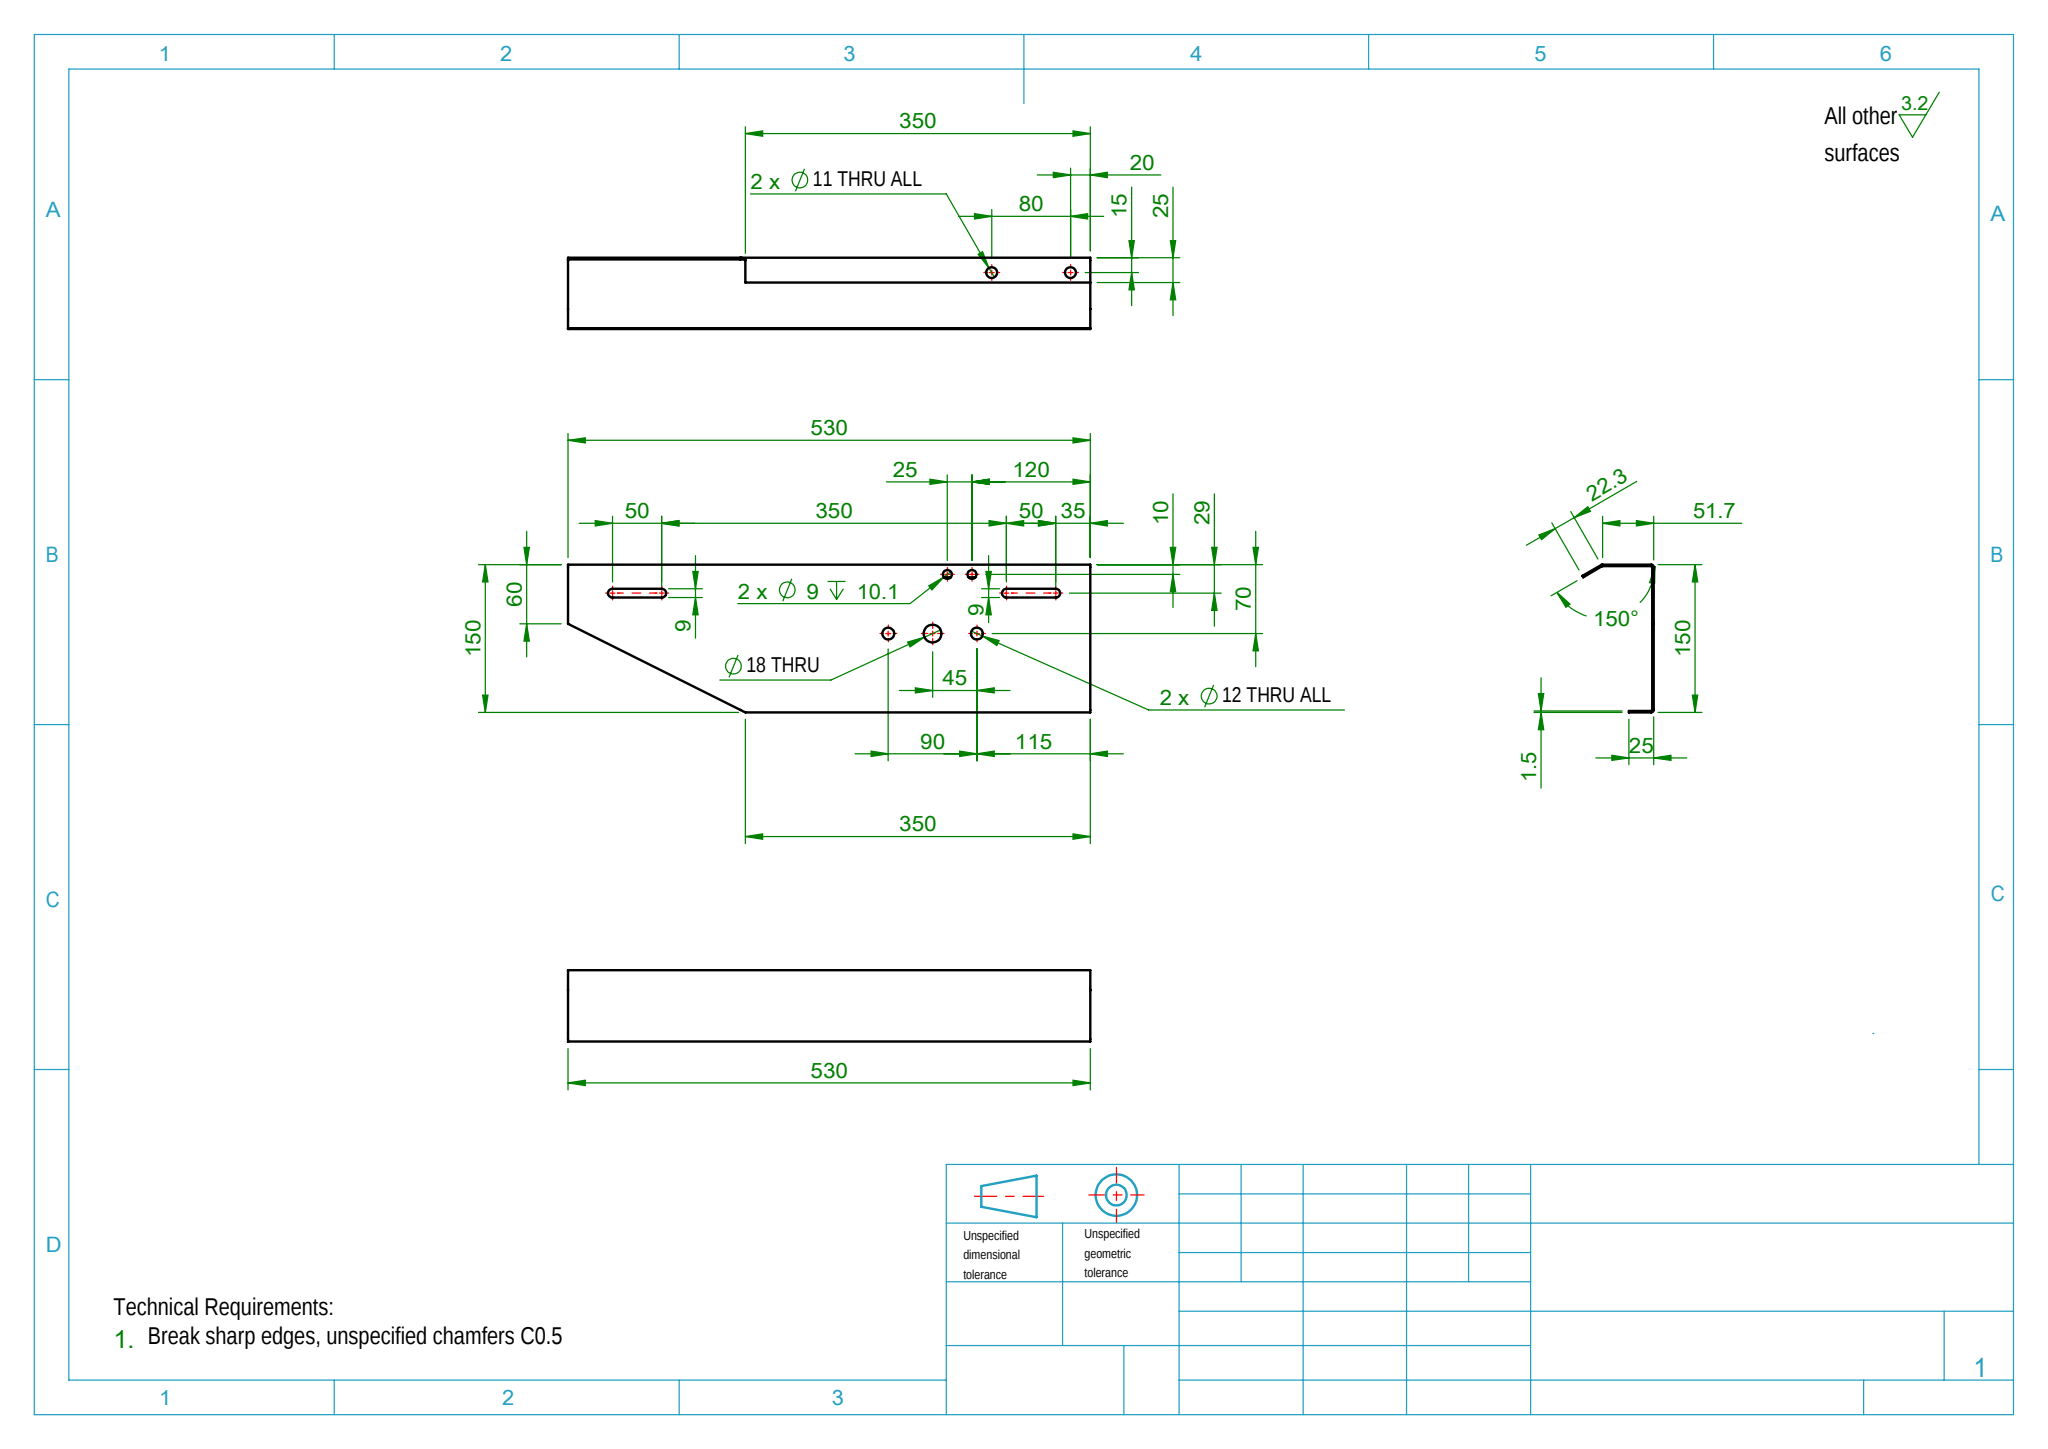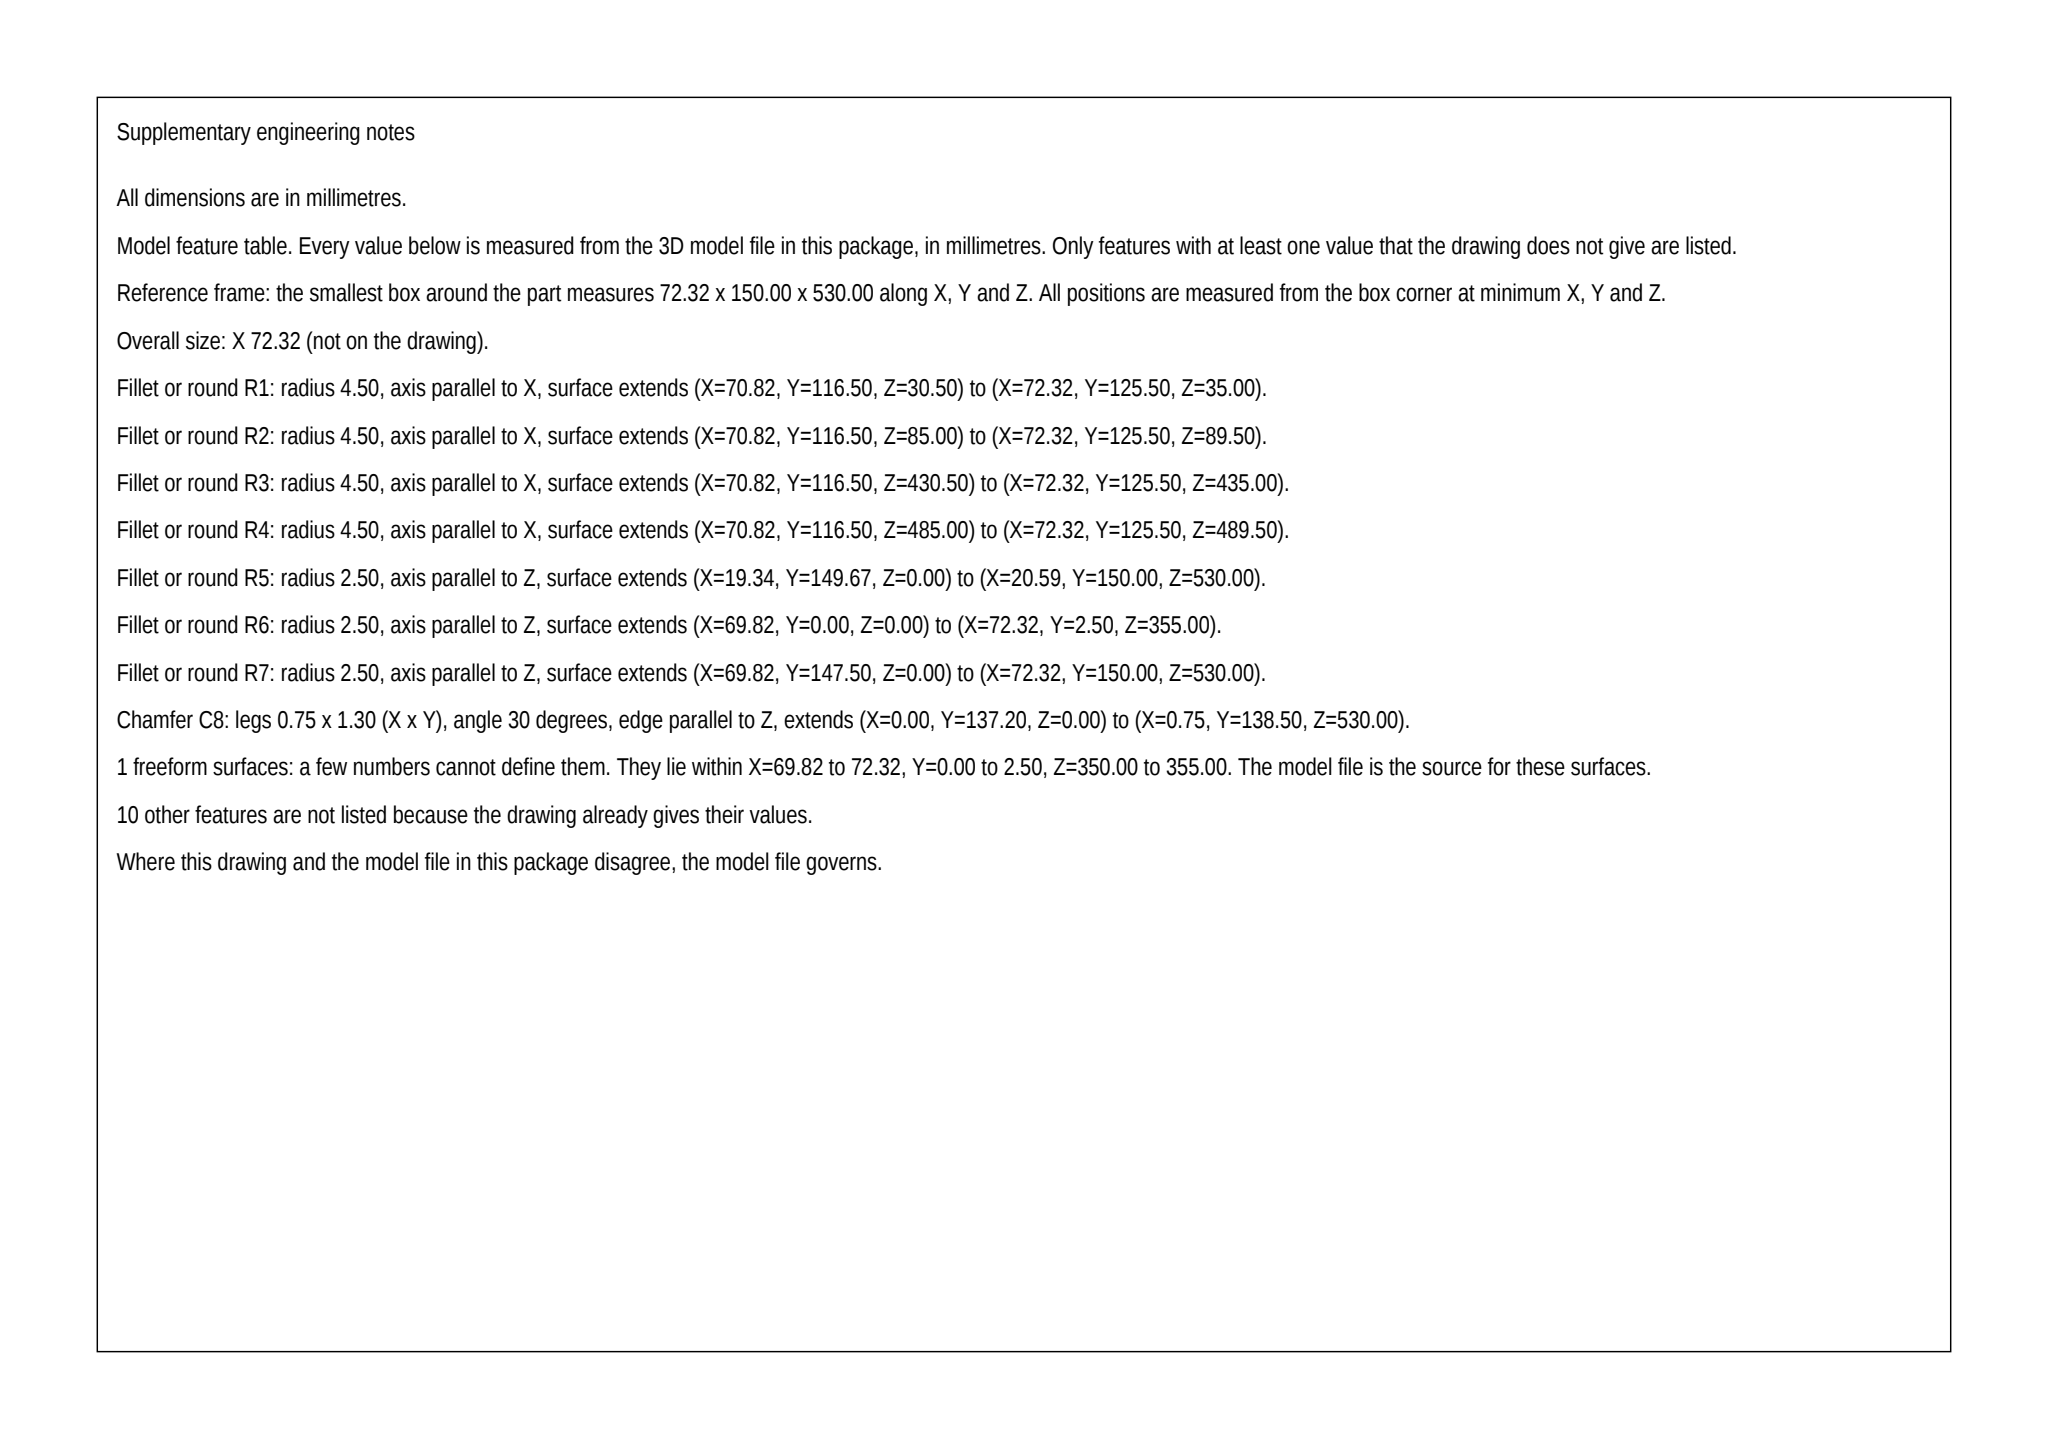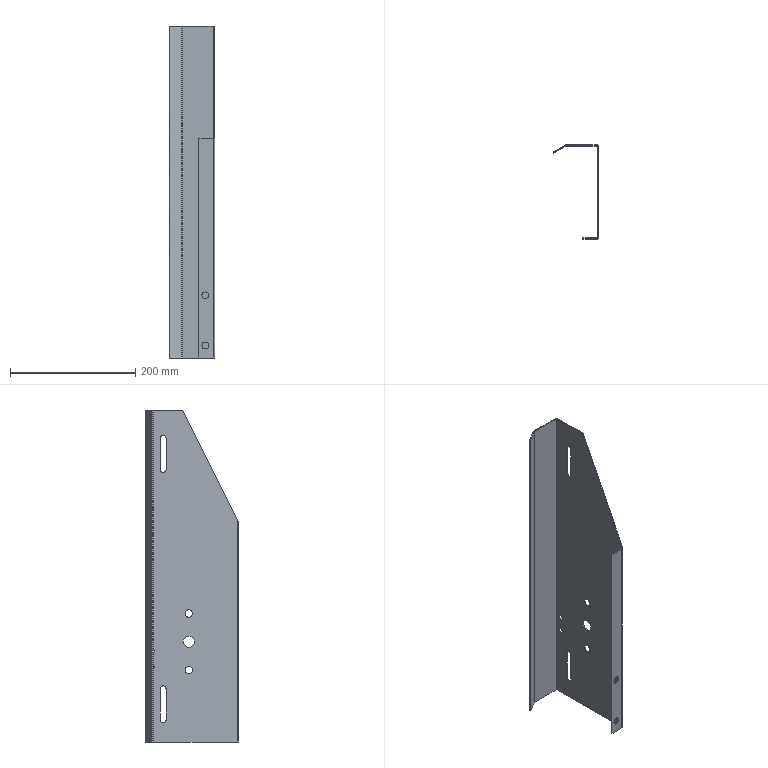Part | SolidWorks | mm | 1 solid | 55 faces | box 72.32 x 150 x 530 mm | volume 174122 mm3 | plane 28 | cylinder 26 | spline 1 | commonest cylinder face diameters 9 x10 11 x4 12 x4 5 x3 2 x3 18 x2
Drawing notes:
DIAG CUT: 90 UP LH END EDGE TO 175 ALONG BOT EDGE | from the solid: Flange/bottom edge cyl L=355 vs part L=530; cut from (z=530,y=90) to (z=355,y=0): run 175, rise 90
2X SLOT 9 WIDE x 59 LG, 50 CTR-CTR, CL 29 FROM TOP EDGE, THRU 1.5 | from the solid: Ø9 x-axis cyls y=121 at z=35&85 and z=435&485, len 1.5; 50 ctr-ctr, 50+9=59 OAL; 150-121=29
Ø18 THRU: 160 FROM RH END, 70 FROM TOP EDGE | from the solid: Ø18 x-axis hole at z=160, y=80; z=0 end is RH (diag cut at z=530 = LH); 150-80=70 from top
ALL BENDS INSIDE R1 (OUTSIDE R2.5), MATL THK 1.5 | from the solid: Coaxial z-axis cyls Ø2 (R1) & Ø5 (R2.5) at (20.59,147.5),(69.82,147.5),(69.82,2.5); plane pairs 1.5 apart